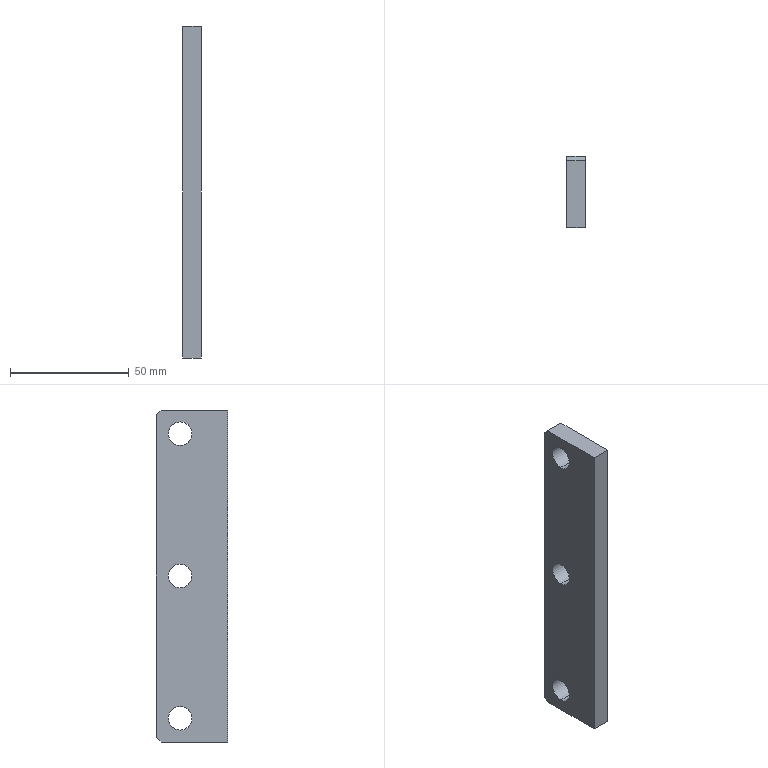Component | SolidWorks | RollerMountingPlate-1 | 1 solid | 14 faces | box 8 x 30 x 140 mm | volume 31683 mm3 | plane 8 | cylinder 6 | commonest cylinder face diameters 10 x6
build123d program:
from build123d import *

# Parameters (mm, degrees)
SKETCH1_W           = 140
SKETCH1_H           = 30
BOSS_EXTRUDE1_DEPTH = 4
SKETCH6_R           = 5
CUT_EXTRUDE11_DEPTH = 73.035
CHAMFER1_SIZE       = 2


with BuildPart() as part:
    # Sketch1 → Boss-Extrude1 (new, symmetric)
    with BuildSketch(Plane.XY):
        Rectangle(SKETCH1_W, SKETCH1_H)
    extrude(amount=BOSS_EXTRUDE1_DEPTH, both=True)

    # Sketch6 → Cut-Extrude11 (cut, through all)
    with BuildSketch(Plane(origin=(0, 0, -4), x_dir=(-1, 0, 0), z_dir=(0, 0, -1))):
        with Locations((0, -5)):
            Circle(SKETCH6_R)
        with Locations((60, -5)):
            Circle(SKETCH6_R)
        with Locations((-60, -5)):
            Circle(SKETCH6_R)
    extrude(amount=-CUT_EXTRUDE11_DEPTH, mode=Mode.SUBTRACT)

    # Chamfer1
    chamfer1_edges = [part.edges().sort_by_distance(p)[0] for p in [
        (70, -15, 0),
        (-70, -15, 0),
    ]]
    chamfer(chamfer1_edges, length=CHAMFER1_SIZE)


solid = part.part

# Placed as in the assembly
solid = solid.moved(Location((119.398, 350.813, 100), (180, 90, 0)))
STEP:
#1=CARTESIAN_POINT('',(4.543,14.008,1.378));
#2=VERTEX_POINT('',#1);
#3=CARTESIAN_POINT('',(4.543,14.008,1.772));
#4=VERTEX_POINT('',#3);
#5=CARTESIAN_POINT('',(4.543,14.008,1.575));
#6=DIRECTION('',(1.,-0.,-0.));
#7=DIRECTION('',(0.,0.,1.));
#8=AXIS2_PLACEMENT_3D('',#5,#6,#7);
#9=CIRCLE('',#8,0.1969);
#10=EDGE_CURVE('',#2,#4,#9,.T.);
#11=ORIENTED_EDGE('',*,*,#10,.F.);
#12=CARTESIAN_POINT('',(4.858,14.008,1.378));
#13=VERTEX_POINT('',#12);
#14=CARTESIAN_POINT('',(4.543,14.008,1.378));
#15=DIRECTION('',(1.,-0.,-0.));
#16=VECTOR('',#15,39.37);
#17=LINE('',#14,#16);
#18=EDGE_CURVE('',#2,#13,#17,.T.);
#19=ORIENTED_EDGE('',*,*,#18,.T.);
#20=CARTESIAN_POINT('',(4.858,14.008,1.772));
#21=VERTEX_POINT('',#20);
#22=CARTESIAN_POINT('',(4.858,14.008,1.575));
#23=DIRECTION('',(1.,-0.,-0.));
#24=DIRECTION('',(0.,0.,1.));
#25=AXIS2_PLACEMENT_3D('',#22,#23,#24);
#26=CIRCLE('',#25,0.1969);
#27=EDGE_CURVE('',#13,#21,#26,.T.);
#28=ORIENTED_EDGE('',*,*,#27,.T.);
#29=CARTESIAN_POINT('',(4.543,14.008,1.772));
#30=DIRECTION('',(1.,-0.,-0.));
#31=VECTOR('',#30,39.37);
#32=LINE('',#29,#31);
#33=EDGE_CURVE('',#4,#21,#32,.T.);
#34=ORIENTED_EDGE('',*,*,#33,.F.);
#35=EDGE_LOOP('',(#11,#19,#28,#34));
#36=FACE_OUTER_BOUND('',#35,.T.);
#37=CARTESIAN_POINT('',(4.543,14.008,1.575));
#38=DIRECTION('',(1.,-0.,-0.));
#39=DIRECTION('',(0.,0.,1.));
#40=AXIS2_PLACEMENT_3D('',#37,#38,#39);
#41=CYLINDRICAL_SURFACE('',#40,0.1969);
#42=ADVANCED_FACE('',(#36),#41,.F.);
#43=CARTESIAN_POINT('',(4.543,14.008,6.102));
#44=VERTEX_POINT('',#43);
#45=CARTESIAN_POINT('',(4.543,14.008,6.496));
#46=VERTEX_POINT('',#45);
#47=CARTESIAN_POINT('',(4.543,14.008,6.299));
#48=DIRECTION('',(1.,-0.,-0.));
#49=DIRECTION('',(0.,0.,1.));
#50=AXIS2_PLACEMENT_3D('',#47,#48,#49);
#51=CIRCLE('',#50,0.1969);
#52=EDGE_CURVE('',#44,#46,#51,.T.);
#53=ORIENTED_EDGE('',*,*,#52,.F.);
#54=CARTESIAN_POINT('',(4.858,14.008,6.102));
#55=VERTEX_POINT('',#54);
#56=CARTESIAN_POINT('',(4.543,14.008,6.102));
#57=DIRECTION('',(1.,-0.,-0.));
#58=VECTOR('',#57,39.37);
#59=LINE('',#56,#58);
#60=EDGE_CURVE('',#44,#55,#59,.T.);
#61=ORIENTED_EDGE('',*,*,#60,.T.);
#62=CARTESIAN_POINT('',(4.858,14.008,6.496));
#63=VERTEX_POINT('',#62);
#64=CARTESIAN_POINT('',(4.858,14.008,6.299));
#65=DIRECTION('',(1.,-0.,-0.));
#66=DIRECTION('',(0.,0.,1.));
#67=AXIS2_PLACEMENT_3D('',#64,#65,#66);
#68=CIRCLE('',#67,0.1969);
#69=EDGE_CURVE('',#55,#63,#68,.T.);
#70=ORIENTED_EDGE('',*,*,#69,.T.);
#71=CARTESIAN_POINT('',(4.543,14.008,6.496));
#72=DIRECTION('',(1.,-0.,-0.));
#73=VECTOR('',#72,39.37);
#74=LINE('',#71,#73);
#75=EDGE_CURVE('',#46,#63,#74,.T.);
#76=ORIENTED_EDGE('',*,*,#75,.F.);
#77=EDGE_LOOP('',(#53,#61,#70,#76));
#78=FACE_OUTER_BOUND('',#77,.T.);
#79=CARTESIAN_POINT('',(4.543,14.008,6.299));
#80=DIRECTION('',(1.,-0.,-0.));
#81=DIRECTION('',(0.,0.,1.));
#82=AXIS2_PLACEMENT_3D('',#79,#80,#81);
#83=CYLINDRICAL_SURFACE('',#82,0.1969);
#84=ADVANCED_FACE('',(#78),#83,.F.);
#85=CARTESIAN_POINT('',(4.543,14.008,3.74));
#86=VERTEX_POINT('',#85);
#87=CARTESIAN_POINT('',(4.543,14.008,4.134));
#88=VERTEX_POINT('',#87);
#89=CARTESIAN_POINT('',(4.543,14.008,3.937));
#90=DIRECTION('',(1.,-0.,-0.));
#91=DIRECTION('',(0.,0.,1.));
#92=AXIS2_PLACEMENT_3D('',#89,#90,#91);
#93=CIRCLE('',#92,0.1969);
#94=EDGE_CURVE('',#86,#88,#93,.T.);
#95=ORIENTED_EDGE('',*,*,#94,.F.);
#96=CARTESIAN_POINT('',(4.858,14.008,3.74));
#97=VERTEX_POINT('',#96);
#98=CARTESIAN_POINT('',(4.543,14.008,3.74));
#99=DIRECTION('',(1.,-0.,-0.));
#100=VECTOR('',#99,39.37);
#101=LINE('',#98,#100);
#102=EDGE_CURVE('',#86,#97,#101,.T.);
#103=ORIENTED_EDGE('',*,*,#102,.T.);
#104=CARTESIAN_POINT('',(4.858,14.008,4.134));
#105=VERTEX_POINT('',#104);
#106=CARTESIAN_POINT('',(4.858,14.008,3.937));
#107=DIRECTION('',(1.,-0.,-0.));
#108=DIRECTION('',(0.,0.,1.));
#109=AXIS2_PLACEMENT_3D('',#106,#107,#108);
#110=CIRCLE('',#109,0.1969);
#111=EDGE_CURVE('',#97,#105,#110,.T.);
#112=ORIENTED_EDGE('',*,*,#111,.T.);
#113=CARTESIAN_POINT('',(4.543,14.008,4.134));
#114=DIRECTION('',(1.,-0.,-0.));
#115=VECTOR('',#114,39.37);
#116=LINE('',#113,#115);
#117=EDGE_CURVE('',#88,#105,#116,.T.);
#118=ORIENTED_EDGE('',*,*,#117,.F.);
#119=EDGE_LOOP('',(#95,#103,#112,#118));
#120=FACE_OUTER_BOUND('',#119,.T.);
#121=CARTESIAN_POINT('',(4.543,14.008,3.937));
#122=DIRECTION('',(1.,-0.,-0.));
#123=DIRECTION('',(0.,0.,1.));
#124=AXIS2_PLACEMENT_3D('',#121,#122,#123);
#125=CYLINDRICAL_SURFACE('',#124,0.1969);
#126=ADVANCED_FACE('',(#120),#125,.F.);
#127=CARTESIAN_POINT('',(4.858,13.221,6.693));
#128=VERTEX_POINT('',#127);
#129=CARTESIAN_POINT('',(4.858,14.323,6.693));
#130=VERTEX_POINT('',#129);
#131=CARTESIAN_POINT('',(4.858,14.402,6.693));
#132=DIRECTION('',(0.,1.,0.));
#133=VECTOR('',#132,39.37);
#134=LINE('',#131,#133);
#135=EDGE_CURVE('',#128,#130,#134,.T.);
#136=ORIENTED_EDGE('',*,*,#135,.T.);
#137=CARTESIAN_POINT('',(4.543,14.323,6.693));
#138=VERTEX_POINT('',#137);
#139=CARTESIAN_POINT('',(4.543,14.323,6.693));
#140=DIRECTION('',(-1.,0.,0.));
#141=VECTOR('',#140,39.37);
#142=LINE('',#139,#141);
#143=EDGE_CURVE('',#130,#138,#142,.T.);
#144=ORIENTED_EDGE('',*,*,#143,.T.);
#145=CARTESIAN_POINT('',(4.543,13.221,6.693));
#146=VERTEX_POINT('',#145);
#147=CARTESIAN_POINT('',(4.543,14.402,6.693));
#148=DIRECTION('',(0.,1.,0.));
#149=VECTOR('',#148,39.37);
#150=LINE('',#147,#149);
#151=EDGE_CURVE('',#146,#138,#150,.T.);
#152=ORIENTED_EDGE('',*,*,#151,.F.);
#153=CARTESIAN_POINT('',(4.543,13.221,6.693));
#154=DIRECTION('',(1.,-0.,-0.));
#155=VECTOR('',#154,39.37);
#156=LINE('',#153,#155);
#157=EDGE_CURVE('',#146,#128,#156,.T.);
#158=ORIENTED_EDGE('',*,*,#157,.T.);
#159=EDGE_LOOP('',(#136,#144,#152,#158));
#160=FACE_OUTER_BOUND('',#159,.T.);
#161=CARTESIAN_POINT('',(4.543,14.402,6.693));
#162=DIRECTION('',(-0.,0.,-1.));
#163=DIRECTION('',(1.,-0.,-0.));
#164=AXIS2_PLACEMENT_3D('',#161,#162,#163);
#165=PLANE('',#164);
#166=ADVANCED_FACE('',(#160),#165,.F.);
#167=CARTESIAN_POINT('',(4.858,14.402,6.614));
#168=VERTEX_POINT('',#167);
#169=CARTESIAN_POINT('',(4.858,14.402,1.26));
#170=VERTEX_POINT('',#169);
#171=CARTESIAN_POINT('',(4.858,14.402,1.181));
#172=DIRECTION('',(-0.,0.,-1.));
#173=VECTOR('',#172,39.37);
#174=LINE('',#171,#173);
#175=EDGE_CURVE('',#168,#170,#174,.T.);
#176=ORIENTED_EDGE('',*,*,#175,.T.);
#177=CARTESIAN_POINT('',(4.543,14.402,1.26));
#178=VERTEX_POINT('',#177);
#179=CARTESIAN_POINT('',(4.543,14.402,1.26));
#180=DIRECTION('',(-1.,0.,0.));
#181=VECTOR('',#180,39.37);
#182=LINE('',#179,#181);
#183=EDGE_CURVE('',#170,#178,#182,.T.);
#184=ORIENTED_EDGE('',*,*,#183,.T.);
#185=CARTESIAN_POINT('',(4.543,14.402,6.614));
#186=VERTEX_POINT('',#185);
#187=CARTESIAN_POINT('',(4.543,14.402,1.181));
#188=DIRECTION('',(-0.,0.,-1.));
#189=VECTOR('',#188,39.37);
#190=LINE('',#187,#189);
#191=EDGE_CURVE('',#186,#178,#190,.T.);
#192=ORIENTED_EDGE('',*,*,#191,.F.);
#193=CARTESIAN_POINT('',(4.543,14.402,6.614));
#194=DIRECTION('',(1.,-0.,-0.));
#195=VECTOR('',#194,39.37);
#196=LINE('',#193,#195);
#197=EDGE_CURVE('',#186,#168,#196,.T.);
#198=ORIENTED_EDGE('',*,*,#197,.T.);
#199=EDGE_LOOP('',(#176,#184,#192,#198));
#200=FACE_OUTER_BOUND('',#199,.T.);
#201=CARTESIAN_POINT('',(4.543,14.402,1.181));
#202=DIRECTION('',(-0.,-1.,-0.));
#203=DIRECTION('',(0.,-0.,1.));
#204=AXIS2_PLACEMENT_3D('',#201,#202,#203);
#205=PLANE('',#204);
#206=ADVANCED_FACE('',(#200),#205,.F.);
#207=CARTESIAN_POINT('',(4.543,14.323,1.181));
#208=VERTEX_POINT('',#207);
#209=CARTESIAN_POINT('',(4.543,13.221,1.181));
#210=VERTEX_POINT('',#209);
#211=CARTESIAN_POINT('',(4.543,14.402,1.181));
#212=DIRECTION('',(-0.,-1.,-0.));
#213=VECTOR('',#212,39.37);
#214=LINE('',#211,#213);
#215=EDGE_CURVE('',#208,#210,#214,.T.);
#216=ORIENTED_EDGE('',*,*,#215,.F.);
#217=CARTESIAN_POINT('',(4.858,14.323,1.181));
#218=VERTEX_POINT('',#217);
#219=CARTESIAN_POINT('',(4.543,14.323,1.181));
#220=DIRECTION('',(1.,-0.,-0.));
#221=VECTOR('',#220,39.37);
#222=LINE('',#219,#221);
#223=EDGE_CURVE('',#208,#218,#222,.T.);
#224=ORIENTED_EDGE('',*,*,#223,.T.);
#225=CARTESIAN_POINT('',(4.858,13.221,1.181));
#226=VERTEX_POINT('',#225);
#227=CARTESIAN_POINT('',(4.858,14.402,1.181));
#228=DIRECTION('',(-0.,-1.,-0.));
#229=VECTOR('',#228,39.37);
#230=LINE('',#227,#229);
#231=EDGE_CURVE('',#218,#226,#230,.T.);
#232=ORIENTED_EDGE('',*,*,#231,.T.);
#233=CARTESIAN_POINT('',(4.543,13.221,1.181));
#234=DIRECTION('',(1.,-0.,-0.));
#235=VECTOR('',#234,39.37);
#236=LINE('',#233,#235);
#237=EDGE_CURVE('',#210,#226,#236,.T.);
#238=ORIENTED_EDGE('',*,*,#237,.F.);
#239=EDGE_LOOP('',(#216,#224,#232,#238));
#240=FACE_OUTER_BOUND('',#239,.T.);
#241=CARTESIAN_POINT('',(4.543,14.402,1.181));
#242=DIRECTION('',(0.,-0.,1.));
#243=DIRECTION('',(-1.,0.,0.));
#244=AXIS2_PLACEMENT_3D('',#241,#242,#243);
#245=PLANE('',#244);
#246=ADVANCED_FACE('',(#240),#245,.F.);
#247=CARTESIAN_POINT('',(4.858,13.221,1.181));
#248=DIRECTION('',(0.,-0.,1.));
#249=VECTOR('',#248,39.37);
#250=LINE('',#247,#249);
#251=EDGE_CURVE('',#226,#128,#250,.T.);
#252=ORIENTED_EDGE('',*,*,#251,.T.);
#253=ORIENTED_EDGE('',*,*,#157,.F.);
#254=CARTESIAN_POINT('',(4.543,13.221,1.181));
#255=DIRECTION('',(0.,-0.,1.));
#256=VECTOR('',#255,39.37);
#257=LINE('',#254,#256);
#258=EDGE_CURVE('',#210,#146,#257,.T.);
#259=ORIENTED_EDGE('',*,*,#258,.F.);
#260=ORIENTED_EDGE('',*,*,#237,.T.);
#261=EDGE_LOOP('',(#252,#253,#259,#260));
#262=FACE_OUTER_BOUND('',#261,.T.);
#263=CARTESIAN_POINT('',(4.543,13.221,1.181));
#264=DIRECTION('',(0.,1.,0.));
#265=DIRECTION('',(-0.,0.,-1.));
#266=AXIS2_PLACEMENT_3D('',#263,#264,#265);
#267=PLANE('',#266);
#268=ADVANCED_FACE('',(#262),#267,.F.);
#269=CARTESIAN_POINT('',(4.543,14.008,1.575));
#270=DIRECTION('',(1.,-0.,-0.));
#271=DIRECTION('',(0.,0.,1.));
#272=AXIS2_PLACEMENT_3D('',#269,#270,#271);
#273=CIRCLE('',#272,0.1969);
#274=EDGE_CURVE('',#4,#2,#273,.T.);
#275=ORIENTED_EDGE('',*,*,#274,.T.);
#276=ORIENTED_EDGE('',*,*,#10,.T.);
#277=EDGE_LOOP('',(#275,#276));
#278=FACE_BOUND('',#277,.T.);
#279=CARTESIAN_POINT('',(4.543,14.008,6.299));
#280=DIRECTION('',(1.,-0.,-0.));
#281=DIRECTION('',(0.,0.,1.));
#282=AXIS2_PLACEMENT_3D('',#279,#280,#281);
#283=CIRCLE('',#282,0.1969);
#284=EDGE_CURVE('',#46,#44,#283,.T.);
#285=ORIENTED_EDGE('',*,*,#284,.T.);
#286=ORIENTED_EDGE('',*,*,#52,.T.);
#287=EDGE_LOOP('',(#285,#286));
#288=FACE_BOUND('',#287,.T.);
#289=CARTESIAN_POINT('',(4.543,14.008,3.937));
#290=DIRECTION('',(1.,-0.,-0.));
#291=DIRECTION('',(0.,0.,1.));
#292=AXIS2_PLACEMENT_3D('',#289,#290,#291);
#293=CIRCLE('',#292,0.1969);
#294=EDGE_CURVE('',#88,#86,#293,.T.);
#295=ORIENTED_EDGE('',*,*,#294,.T.);
#296=ORIENTED_EDGE('',*,*,#94,.T.);
#297=EDGE_LOOP('',(#295,#296));
#298=FACE_BOUND('',#297,.T.);
#299=ORIENTED_EDGE('',*,*,#191,.T.);
#300=CARTESIAN_POINT('',(4.543,15.445,2.303));
#301=DIRECTION('',(-0.,-0.7071,-0.7071));
#302=VECTOR('',#301,39.37);
#303=LINE('',#300,#302);
#304=EDGE_CURVE('',#178,#208,#303,.T.);
#305=ORIENTED_EDGE('',*,*,#304,.T.);
#306=ORIENTED_EDGE('',*,*,#215,.T.);
#307=ORIENTED_EDGE('',*,*,#258,.T.);
#308=ORIENTED_EDGE('',*,*,#151,.T.);
#309=CARTESIAN_POINT('',(4.543,15.445,5.571));
#310=DIRECTION('',(0.,0.7071,-0.7071));
#311=VECTOR('',#310,39.37);
#312=LINE('',#309,#311);
#313=EDGE_CURVE('',#138,#186,#312,.T.);
#314=ORIENTED_EDGE('',*,*,#313,.T.);
#315=EDGE_LOOP('',(#299,#305,#306,#307,#308,#314));
#316=FACE_OUTER_BOUND('',#315,.T.);
#317=CARTESIAN_POINT('',(4.543,13.812,3.937));
#318=DIRECTION('',(-1.,0.,0.));
#319=DIRECTION('',(-0.,0.,-1.));
#320=AXIS2_PLACEMENT_3D('',#317,#318,#319);
#321=PLANE('',#320);
#322=ADVANCED_FACE('',(#278,#288,#298,#316),#321,.T.);
#323=CARTESIAN_POINT('',(4.858,14.008,1.575));
#324=DIRECTION('',(1.,-0.,-0.));
#325=DIRECTION('',(0.,0.,1.));
#326=AXIS2_PLACEMENT_3D('',#323,#324,#325);
#327=CIRCLE('',#326,0.1969);
#328=EDGE_CURVE('',#21,#13,#327,.T.);
#329=ORIENTED_EDGE('',*,*,#328,.F.);
#330=ORIENTED_EDGE('',*,*,#27,.F.);
#331=EDGE_LOOP('',(#329,#330));
#332=FACE_BOUND('',#331,.T.);
#333=CARTESIAN_POINT('',(4.858,14.008,6.299));
#334=DIRECTION('',(1.,-0.,-0.));
#335=DIRECTION('',(0.,0.,1.));
#336=AXIS2_PLACEMENT_3D('',#333,#334,#335);
#337=CIRCLE('',#336,0.1969);
#338=EDGE_CURVE('',#63,#55,#337,.T.);
#339=ORIENTED_EDGE('',*,*,#338,.F.);
#340=ORIENTED_EDGE('',*,*,#69,.F.);
#341=EDGE_LOOP('',(#339,#340));
#342=FACE_BOUND('',#341,.T.);
#343=CARTESIAN_POINT('',(4.858,14.008,3.937));
#344=DIRECTION('',(1.,-0.,-0.));
#345=DIRECTION('',(0.,0.,1.));
#346=AXIS2_PLACEMENT_3D('',#343,#344,#345);
#347=CIRCLE('',#346,0.1969);
#348=EDGE_CURVE('',#105,#97,#347,.T.);
#349=ORIENTED_EDGE('',*,*,#348,.F.);
#350=ORIENTED_EDGE('',*,*,#111,.F.);
#351=EDGE_LOOP('',(#349,#350));
#352=FACE_BOUND('',#351,.T.);
#353=ORIENTED_EDGE('',*,*,#231,.F.);
#354=CARTESIAN_POINT('',(4.858,14.323,1.181));
#355=DIRECTION('',(0.,0.7071,0.7071));
#356=VECTOR('',#355,39.37);
#357=LINE('',#354,#356);
#358=EDGE_CURVE('',#218,#170,#357,.T.);
#359=ORIENTED_EDGE('',*,*,#358,.T.);
#360=ORIENTED_EDGE('',*,*,#175,.F.);
#361=CARTESIAN_POINT('',(4.858,14.402,6.614));
#362=DIRECTION('',(-0.,-0.7071,0.7071));
#363=VECTOR('',#362,39.37);
#364=LINE('',#361,#363);
#365=EDGE_CURVE('',#168,#130,#364,.T.);
#366=ORIENTED_EDGE('',*,*,#365,.T.);
#367=ORIENTED_EDGE('',*,*,#135,.F.);
#368=ORIENTED_EDGE('',*,*,#251,.F.);
#369=EDGE_LOOP('',(#353,#359,#360,#366,#367,#368));
#370=FACE_OUTER_BOUND('',#369,.T.);
#371=CARTESIAN_POINT('',(4.858,13.812,3.937));
#372=DIRECTION('',(-1.,0.,0.));
#373=DIRECTION('',(-0.,0.,-1.));
#374=AXIS2_PLACEMENT_3D('',#371,#372,#373);
#375=PLANE('',#374);
#376=ADVANCED_FACE('',(#332,#342,#352,#370),#375,.F.);
#377=ORIENTED_EDGE('',*,*,#102,.F.);
#378=ORIENTED_EDGE('',*,*,#294,.F.);
#379=ORIENTED_EDGE('',*,*,#117,.T.);
#380=ORIENTED_EDGE('',*,*,#348,.T.);
#381=EDGE_LOOP('',(#377,#378,#379,#380));
#382=FACE_OUTER_BOUND('',#381,.T.);
#383=CARTESIAN_POINT('',(4.543,14.008,3.937));
#384=DIRECTION('',(1.,-0.,-0.));
#385=DIRECTION('',(0.,0.,1.));
#386=AXIS2_PLACEMENT_3D('',#383,#384,#385);
#387=CYLINDRICAL_SURFACE('',#386,0.1969);
#388=ADVANCED_FACE('',(#382),#387,.F.);
#389=ORIENTED_EDGE('',*,*,#60,.F.);
#390=ORIENTED_EDGE('',*,*,#284,.F.);
#391=ORIENTED_EDGE('',*,*,#75,.T.);
#392=ORIENTED_EDGE('',*,*,#338,.T.);
#393=EDGE_LOOP('',(#389,#390,#391,#392));
#394=FACE_OUTER_BOUND('',#393,.T.);
#395=CARTESIAN_POINT('',(4.543,14.008,6.299));
#396=DIRECTION('',(1.,-0.,-0.));
#397=DIRECTION('',(0.,0.,1.));
#398=AXIS2_PLACEMENT_3D('',#395,#396,#397);
#399=CYLINDRICAL_SURFACE('',#398,0.1969);
#400=ADVANCED_FACE('',(#394),#399,.F.);
#401=ORIENTED_EDGE('',*,*,#18,.F.);
#402=ORIENTED_EDGE('',*,*,#274,.F.);
#403=ORIENTED_EDGE('',*,*,#33,.T.);
#404=ORIENTED_EDGE('',*,*,#328,.T.);
#405=EDGE_LOOP('',(#401,#402,#403,#404));
#406=FACE_OUTER_BOUND('',#405,.T.);
#407=CARTESIAN_POINT('',(4.543,14.008,1.575));
#408=DIRECTION('',(1.,-0.,-0.));
#409=DIRECTION('',(0.,0.,1.));
#410=AXIS2_PLACEMENT_3D('',#407,#408,#409);
#411=CYLINDRICAL_SURFACE('',#410,0.1969);
#412=ADVANCED_FACE('',(#406),#411,.F.);
#413=ORIENTED_EDGE('',*,*,#304,.F.);
#414=ORIENTED_EDGE('',*,*,#183,.F.);
#415=ORIENTED_EDGE('',*,*,#358,.F.);
#416=ORIENTED_EDGE('',*,*,#223,.F.);
#417=EDGE_LOOP('',(#413,#414,#415,#416));
#418=FACE_OUTER_BOUND('',#417,.T.);
#419=CARTESIAN_POINT('',(4.543,14.323,1.181));
#420=DIRECTION('',(-0.,-0.7071,0.7071));
#421=DIRECTION('',(1.,-0.,-0.));
#422=AXIS2_PLACEMENT_3D('',#419,#420,#421);
#423=PLANE('',#422);
#424=ADVANCED_FACE('',(#418),#423,.F.);
#425=ORIENTED_EDGE('',*,*,#313,.F.);
#426=ORIENTED_EDGE('',*,*,#143,.F.);
#427=ORIENTED_EDGE('',*,*,#365,.F.);
#428=ORIENTED_EDGE('',*,*,#197,.F.);
#429=EDGE_LOOP('',(#425,#426,#427,#428));
#430=FACE_OUTER_BOUND('',#429,.T.);
#431=CARTESIAN_POINT('',(4.543,14.402,6.614));
#432=DIRECTION('',(-0.,-0.7071,-0.7071));
#433=DIRECTION('',(1.,-0.,-0.));
#434=AXIS2_PLACEMENT_3D('',#431,#432,#433);
#435=PLANE('',#434);
#436=ADVANCED_FACE('',(#430),#435,.F.);
#437=CLOSED_SHELL('',(#42,#84,#126,#166,#206,#246,#268,#322,#376,#388,#400,#412,#424,#436));
#438=MANIFOLD_SOLID_BREP('',#437);
#439=CARTESIAN_POINT('',(0.,0.,0.));
#440=DIRECTION('',(0.,0.,1.));
#441=DIRECTION('',(1.,0.,0.));
#442=AXIS2_PLACEMENT_3D('',#439,#440,#441);
#443=(LENGTH_UNIT()NAMED_UNIT(*)SI_UNIT($,.METRE.));
#444=LENGTH_MEASURE_WITH_UNIT(LENGTH_MEASURE(0.0254),#443);
#445=DIMENSIONAL_EXPONENTS(1.,0.,0.,0.,0.,0.,0.);
#446=(CONVERSION_BASED_UNIT('',#444)LENGTH_UNIT()NAMED_UNIT(#445));
#447=UNCERTAINTY_MEASURE_WITH_UNIT(LENGTH_MEASURE(0.00001),#446,'','');
#448=(NAMED_UNIT(*)PLANE_ANGLE_UNIT()SI_UNIT($,.RADIAN.));
#449=(NAMED_UNIT(*)SI_UNIT($,.STERADIAN.)SOLID_ANGLE_UNIT());
#450=(GEOMETRIC_REPRESENTATION_CONTEXT(3)GLOBAL_UNCERTAINTY_ASSIGNED_CONTEXT((#447))GLOBAL_UNIT_ASSIGNED_CONTEXT((#446,#448,#449))REPRESENTATION_CONTEXT('',''));
#451=ADVANCED_BREP_SHAPE_REPRESENTATION('',(#438,#442),#450);
#452=COLOUR_RGB('',0.7922,0.8196,0.9333);
#453=FILL_AREA_STYLE_COLOUR('',#452);
#454=FILL_AREA_STYLE('',(#453));
#455=SURFACE_STYLE_FILL_AREA(#454);
#456=SURFACE_SIDE_STYLE('',(#455));
#457=SURFACE_STYLE_USAGE(.BOTH.,#456);
#458=PRESENTATION_STYLE_ASSIGNMENT((#457));
#459=STYLED_ITEM('',(#458),#438);
#460=PRESENTATION_LAYER_ASSIGNMENT('','',(#459));
#461=(LENGTH_UNIT()NAMED_UNIT(*)SI_UNIT($,.METRE.));
#462=LENGTH_MEASURE_WITH_UNIT(LENGTH_MEASURE(0.0254),#461);
#463=DIMENSIONAL_EXPONENTS(1.,0.,0.,0.,0.,0.,0.);
#464=(CONVERSION_BASED_UNIT('',#462)LENGTH_UNIT()NAMED_UNIT(#463));
#465=UNCERTAINTY_MEASURE_WITH_UNIT(LENGTH_MEASURE(0.00001),#464,'','');
#466=(NAMED_UNIT(*)PLANE_ANGLE_UNIT()SI_UNIT($,.RADIAN.));
#467=(NAMED_UNIT(*)SI_UNIT($,.STERADIAN.)SOLID_ANGLE_UNIT());
#468=(GEOMETRIC_REPRESENTATION_CONTEXT(3)GLOBAL_UNCERTAINTY_ASSIGNED_CONTEXT((#465))GLOBAL_UNIT_ASSIGNED_CONTEXT((#464,#466,#467))REPRESENTATION_CONTEXT('',''));
#469=MECHANICAL_DESIGN_GEOMETRIC_PRESENTATION_REPRESENTATION('',(#459),#468);